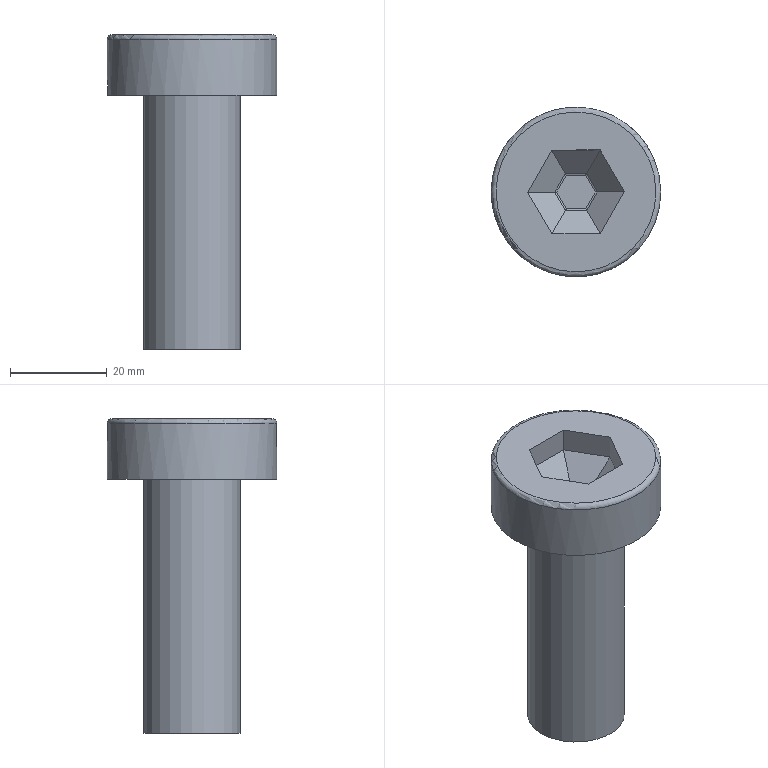Component | NX | A_HEX_SCREW | 1 solid | 25 faces | volume 26504 mm3 | plane 16 | cylinder 8 | torus 1 | commonest cylinder face diameters 1 x6 35 x1 20 x1